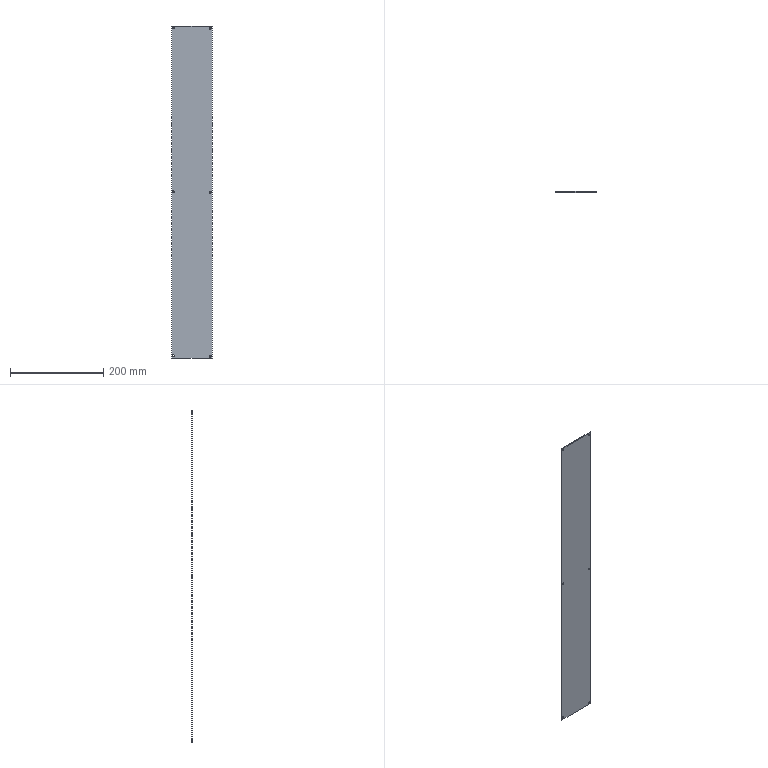Component | SolidWorks | ElectricalBoxCoverPlate2-1 | 1 solid | 18 faces | box 88 x 2 x 713 mm | volume 125337 mm3 | cylinder 12 | plane 6 | commonest cylinder face diameters 4 x12
build123d program:
from build123d import *

# Parameters (mm, degrees)
SKETCH1_W           = 713
SKETCH1_H           = 88
BOSS_EXTRUDE1_DEPTH = 2
SKETCH2_R           = 2
CUT_EXTRUDE1_DEPTH  = 2
LPATTERN1_COUNT     = 3
LPATTERN1_PITCH     = 352


with BuildPart() as part:
    # Sketch1 → Boss-Extrude1 (new body)
    with BuildSketch(Plane.XY):
        with Locations((280.981, -8.624)):
            Rectangle(SKETCH1_W, SKETCH1_H)
    extrude(amount=BOSS_EXTRUDE1_DEPTH)

    # Sketch2 → Cut-Extrude1 (cut)
    with BuildSketch(Plane.XY.offset(2)):
        with Locations((-71.519, 31.376)):
            Circle(SKETCH2_R)
        with Locations((-70.519, -47.624)):
            Circle(SKETCH2_R)
    cut_extrude1 = extrude(amount=-CUT_EXTRUDE1_DEPTH, mode=Mode.SUBTRACT)

    # LPattern1: Cut-Extrude1 ×3
    with Locations(*[(i * LPATTERN1_PITCH, 0, 0) for i in range(1, LPATTERN1_COUNT)]):
        add(cut_extrude1, mode=Mode.SUBTRACT)


solid = part.part

# Placed as in the assembly
solid = solid.moved(Location((311.826, 539.566, 414.962), (-90, 0, 90)))
STEP:
#1=COLOUR_RGB('',0.7922,0.8196,0.9333);
#2=FILL_AREA_STYLE_COLOUR('',#1);
#3=FILL_AREA_STYLE('',(#2));
#4=SURFACE_STYLE_FILL_AREA(#3);
#5=SURFACE_SIDE_STYLE('',(#4));
#6=SURFACE_STYLE_USAGE(.BOTH.,#5);
#7=PRESENTATION_STYLE_ASSIGNMENT((#6));
#8=CARTESIAN_POINT('',(14.152,21.243,-8.524));
#9=VERTEX_POINT('',#8);
#10=CARTESIAN_POINT('',(14.152,21.243,-8.682));
#11=VERTEX_POINT('',#10);
#12=CARTESIAN_POINT('',(14.152,21.243,-8.603));
#13=DIRECTION('',(0.,1.,0.));
#14=DIRECTION('',(0.,0.,-1.));
#15=AXIS2_PLACEMENT_3D('',#12,#13,#14);
#16=CIRCLE('',#15,0.07874);
#17=EDGE_CURVE('',#9,#11,#16,.T.);
#18=ORIENTED_EDGE('',*,*,#17,.F.);
#19=CARTESIAN_POINT('',(14.152,21.322,-8.524));
#20=VERTEX_POINT('',#19);
#21=CARTESIAN_POINT('',(14.152,21.243,-8.524));
#22=DIRECTION('',(0.,1.,0.));
#23=VECTOR('',#22,39.37);
#24=LINE('',#21,#23);
#25=EDGE_CURVE('',#9,#20,#24,.T.);
#26=ORIENTED_EDGE('',*,*,#25,.T.);
#27=CARTESIAN_POINT('',(14.152,21.322,-8.682));
#28=VERTEX_POINT('',#27);
#29=CARTESIAN_POINT('',(14.152,21.322,-8.603));
#30=DIRECTION('',(0.,1.,0.));
#31=DIRECTION('',(0.,0.,-1.));
#32=AXIS2_PLACEMENT_3D('',#29,#30,#31);
#33=CIRCLE('',#32,0.07874);
#34=EDGE_CURVE('',#20,#28,#33,.T.);
#35=ORIENTED_EDGE('',*,*,#34,.T.);
#36=CARTESIAN_POINT('',(14.152,21.243,-8.682));
#37=DIRECTION('',(0.,1.,0.));
#38=VECTOR('',#37,39.37);
#39=LINE('',#36,#38);
#40=EDGE_CURVE('',#11,#28,#39,.T.);
#41=ORIENTED_EDGE('',*,*,#40,.F.);
#42=EDGE_LOOP('',(#18,#26,#35,#41));
#43=FACE_OUTER_BOUND('',#42,.T.);
#44=CARTESIAN_POINT('',(14.152,21.243,-8.603));
#45=DIRECTION('',(0.,1.,0.));
#46=DIRECTION('',(0.,0.,-1.));
#47=AXIS2_PLACEMENT_3D('',#44,#45,#46);
#48=CYLINDRICAL_SURFACE('',#47,0.07874);
#49=ADVANCED_FACE('',(#43),#48,.F.);
#50=CARTESIAN_POINT('',(11.041,21.243,-8.485));
#51=VERTEX_POINT('',#50);
#52=CARTESIAN_POINT('',(11.041,21.243,-8.642));
#53=VERTEX_POINT('',#52);
#54=CARTESIAN_POINT('',(11.041,21.243,-8.564));
#55=DIRECTION('',(0.,1.,0.));
#56=DIRECTION('',(0.,0.,-1.));
#57=AXIS2_PLACEMENT_3D('',#54,#55,#56);
#58=CIRCLE('',#57,0.07874);
#59=EDGE_CURVE('',#51,#53,#58,.T.);
#60=ORIENTED_EDGE('',*,*,#59,.F.);
#61=CARTESIAN_POINT('',(11.041,21.322,-8.485));
#62=VERTEX_POINT('',#61);
#63=CARTESIAN_POINT('',(11.041,21.243,-8.485));
#64=DIRECTION('',(0.,1.,0.));
#65=VECTOR('',#64,39.37);
#66=LINE('',#63,#65);
#67=EDGE_CURVE('',#51,#62,#66,.T.);
#68=ORIENTED_EDGE('',*,*,#67,.T.);
#69=CARTESIAN_POINT('',(11.041,21.322,-8.642));
#70=VERTEX_POINT('',#69);
#71=CARTESIAN_POINT('',(11.041,21.322,-8.564));
#72=DIRECTION('',(0.,1.,0.));
#73=DIRECTION('',(0.,0.,-1.));
#74=AXIS2_PLACEMENT_3D('',#71,#72,#73);
#75=CIRCLE('',#74,0.07874);
#76=EDGE_CURVE('',#62,#70,#75,.T.);
#77=ORIENTED_EDGE('',*,*,#76,.T.);
#78=CARTESIAN_POINT('',(11.041,21.243,-8.642));
#79=DIRECTION('',(0.,1.,0.));
#80=VECTOR('',#79,39.37);
#81=LINE('',#78,#80);
#82=EDGE_CURVE('',#53,#70,#81,.T.);
#83=ORIENTED_EDGE('',*,*,#82,.F.);
#84=EDGE_LOOP('',(#60,#68,#77,#83));
#85=FACE_OUTER_BOUND('',#84,.T.);
#86=CARTESIAN_POINT('',(11.041,21.243,-8.564));
#87=DIRECTION('',(0.,1.,0.));
#88=DIRECTION('',(0.,0.,-1.));
#89=AXIS2_PLACEMENT_3D('',#86,#87,#88);
#90=CYLINDRICAL_SURFACE('',#89,0.07874);
#91=ADVANCED_FACE('',(#85),#90,.F.);
#92=CARTESIAN_POINT('',(14.152,21.243,5.334));
#93=VERTEX_POINT('',#92);
#94=CARTESIAN_POINT('',(14.152,21.243,5.176));
#95=VERTEX_POINT('',#94);
#96=CARTESIAN_POINT('',(14.152,21.243,5.255));
#97=DIRECTION('',(0.,1.,0.));
#98=DIRECTION('',(0.,0.,-1.));
#99=AXIS2_PLACEMENT_3D('',#96,#97,#98);
#100=CIRCLE('',#99,0.07874);
#101=EDGE_CURVE('',#93,#95,#100,.T.);
#102=ORIENTED_EDGE('',*,*,#101,.F.);
#103=CARTESIAN_POINT('',(14.152,21.322,5.334));
#104=VERTEX_POINT('',#103);
#105=CARTESIAN_POINT('',(14.152,21.243,5.334));
#106=DIRECTION('',(0.,1.,0.));
#107=VECTOR('',#106,39.37);
#108=LINE('',#105,#107);
#109=EDGE_CURVE('',#93,#104,#108,.T.);
#110=ORIENTED_EDGE('',*,*,#109,.T.);
#111=CARTESIAN_POINT('',(14.152,21.322,5.176));
#112=VERTEX_POINT('',#111);
#113=CARTESIAN_POINT('',(14.152,21.322,5.255));
#114=DIRECTION('',(0.,1.,0.));
#115=DIRECTION('',(0.,0.,-1.));
#116=AXIS2_PLACEMENT_3D('',#113,#114,#115);
#117=CIRCLE('',#116,0.07874);
#118=EDGE_CURVE('',#104,#112,#117,.T.);
#119=ORIENTED_EDGE('',*,*,#118,.T.);
#120=CARTESIAN_POINT('',(14.152,21.243,5.176));
#121=DIRECTION('',(0.,1.,0.));
#122=VECTOR('',#121,39.37);
#123=LINE('',#120,#122);
#124=EDGE_CURVE('',#95,#112,#123,.T.);
#125=ORIENTED_EDGE('',*,*,#124,.F.);
#126=EDGE_LOOP('',(#102,#110,#119,#125));
#127=FACE_OUTER_BOUND('',#126,.T.);
#128=CARTESIAN_POINT('',(14.152,21.243,5.255));
#129=DIRECTION('',(0.,1.,0.));
#130=DIRECTION('',(0.,0.,-1.));
#131=AXIS2_PLACEMENT_3D('',#128,#129,#130);
#132=CYLINDRICAL_SURFACE('',#131,0.07874);
#133=ADVANCED_FACE('',(#127),#132,.F.);
#134=CARTESIAN_POINT('',(11.041,21.243,5.373));
#135=VERTEX_POINT('',#134);
#136=CARTESIAN_POINT('',(11.041,21.243,5.216));
#137=VERTEX_POINT('',#136);
#138=CARTESIAN_POINT('',(11.041,21.243,5.295));
#139=DIRECTION('',(0.,1.,0.));
#140=DIRECTION('',(0.,0.,-1.));
#141=AXIS2_PLACEMENT_3D('',#138,#139,#140);
#142=CIRCLE('',#141,0.07874);
#143=EDGE_CURVE('',#135,#137,#142,.T.);
#144=ORIENTED_EDGE('',*,*,#143,.F.);
#145=CARTESIAN_POINT('',(11.041,21.322,5.373));
#146=VERTEX_POINT('',#145);
#147=CARTESIAN_POINT('',(11.041,21.243,5.373));
#148=DIRECTION('',(0.,1.,0.));
#149=VECTOR('',#148,39.37);
#150=LINE('',#147,#149);
#151=EDGE_CURVE('',#135,#146,#150,.T.);
#152=ORIENTED_EDGE('',*,*,#151,.T.);
#153=CARTESIAN_POINT('',(11.041,21.322,5.216));
#154=VERTEX_POINT('',#153);
#155=CARTESIAN_POINT('',(11.041,21.322,5.295));
#156=DIRECTION('',(0.,1.,0.));
#157=DIRECTION('',(0.,0.,-1.));
#158=AXIS2_PLACEMENT_3D('',#155,#156,#157);
#159=CIRCLE('',#158,0.07874);
#160=EDGE_CURVE('',#146,#154,#159,.T.);
#161=ORIENTED_EDGE('',*,*,#160,.T.);
#162=CARTESIAN_POINT('',(11.041,21.243,5.216));
#163=DIRECTION('',(0.,1.,0.));
#164=VECTOR('',#163,39.37);
#165=LINE('',#162,#164);
#166=EDGE_CURVE('',#137,#154,#165,.T.);
#167=ORIENTED_EDGE('',*,*,#166,.F.);
#168=EDGE_LOOP('',(#144,#152,#161,#167));
#169=FACE_OUTER_BOUND('',#168,.T.);
#170=CARTESIAN_POINT('',(11.041,21.243,5.295));
#171=DIRECTION('',(0.,1.,0.));
#172=DIRECTION('',(0.,0.,-1.));
#173=AXIS2_PLACEMENT_3D('',#170,#171,#172);
#174=CYLINDRICAL_SURFACE('',#173,0.07874);
#175=ADVANCED_FACE('',(#169),#174,.F.);
#176=CARTESIAN_POINT('',(14.152,21.243,19.192));
#177=VERTEX_POINT('',#176);
#178=CARTESIAN_POINT('',(14.152,21.243,19.035));
#179=VERTEX_POINT('',#178);
#180=CARTESIAN_POINT('',(14.152,21.243,19.113));
#181=DIRECTION('',(0.,1.,0.));
#182=DIRECTION('',(0.,0.,-1.));
#183=AXIS2_PLACEMENT_3D('',#180,#181,#182);
#184=CIRCLE('',#183,0.07874);
#185=EDGE_CURVE('',#177,#179,#184,.T.);
#186=ORIENTED_EDGE('',*,*,#185,.F.);
#187=CARTESIAN_POINT('',(14.152,21.322,19.192));
#188=VERTEX_POINT('',#187);
#189=CARTESIAN_POINT('',(14.152,21.243,19.192));
#190=DIRECTION('',(0.,1.,0.));
#191=VECTOR('',#190,39.37);
#192=LINE('',#189,#191);
#193=EDGE_CURVE('',#177,#188,#192,.T.);
#194=ORIENTED_EDGE('',*,*,#193,.T.);
#195=CARTESIAN_POINT('',(14.152,21.322,19.035));
#196=VERTEX_POINT('',#195);
#197=CARTESIAN_POINT('',(14.152,21.322,19.113));
#198=DIRECTION('',(0.,1.,0.));
#199=DIRECTION('',(0.,0.,-1.));
#200=AXIS2_PLACEMENT_3D('',#197,#198,#199);
#201=CIRCLE('',#200,0.07874);
#202=EDGE_CURVE('',#188,#196,#201,.T.);
#203=ORIENTED_EDGE('',*,*,#202,.T.);
#204=CARTESIAN_POINT('',(14.152,21.243,19.035));
#205=DIRECTION('',(0.,1.,0.));
#206=VECTOR('',#205,39.37);
#207=LINE('',#204,#206);
#208=EDGE_CURVE('',#179,#196,#207,.T.);
#209=ORIENTED_EDGE('',*,*,#208,.F.);
#210=EDGE_LOOP('',(#186,#194,#203,#209));
#211=FACE_OUTER_BOUND('',#210,.T.);
#212=CARTESIAN_POINT('',(14.152,21.243,19.113));
#213=DIRECTION('',(0.,1.,0.));
#214=DIRECTION('',(0.,0.,-1.));
#215=AXIS2_PLACEMENT_3D('',#212,#213,#214);
#216=CYLINDRICAL_SURFACE('',#215,0.07874);
#217=ADVANCED_FACE('',(#211),#216,.F.);
#218=CARTESIAN_POINT('',(11.041,21.243,19.232));
#219=VERTEX_POINT('',#218);
#220=CARTESIAN_POINT('',(11.041,21.243,19.074));
#221=VERTEX_POINT('',#220);
#222=CARTESIAN_POINT('',(11.041,21.243,19.153));
#223=DIRECTION('',(0.,1.,0.));
#224=DIRECTION('',(0.,0.,-1.));
#225=AXIS2_PLACEMENT_3D('',#222,#223,#224);
#226=CIRCLE('',#225,0.07874);
#227=EDGE_CURVE('',#219,#221,#226,.T.);
#228=ORIENTED_EDGE('',*,*,#227,.F.);
#229=CARTESIAN_POINT('',(11.041,21.322,19.232));
#230=VERTEX_POINT('',#229);
#231=CARTESIAN_POINT('',(11.041,21.243,19.232));
#232=DIRECTION('',(0.,1.,0.));
#233=VECTOR('',#232,39.37);
#234=LINE('',#231,#233);
#235=EDGE_CURVE('',#219,#230,#234,.T.);
#236=ORIENTED_EDGE('',*,*,#235,.T.);
#237=CARTESIAN_POINT('',(11.041,21.322,19.074));
#238=VERTEX_POINT('',#237);
#239=CARTESIAN_POINT('',(11.041,21.322,19.153));
#240=DIRECTION('',(0.,1.,0.));
#241=DIRECTION('',(0.,0.,-1.));
#242=AXIS2_PLACEMENT_3D('',#239,#240,#241);
#243=CIRCLE('',#242,0.07874);
#244=EDGE_CURVE('',#230,#238,#243,.T.);
#245=ORIENTED_EDGE('',*,*,#244,.T.);
#246=CARTESIAN_POINT('',(11.041,21.243,19.074));
#247=DIRECTION('',(0.,1.,0.));
#248=VECTOR('',#247,39.37);
#249=LINE('',#246,#248);
#250=EDGE_CURVE('',#221,#238,#249,.T.);
#251=ORIENTED_EDGE('',*,*,#250,.F.);
#252=EDGE_LOOP('',(#228,#236,#245,#251));
#253=FACE_OUTER_BOUND('',#252,.T.);
#254=CARTESIAN_POINT('',(11.041,21.243,19.153));
#255=DIRECTION('',(0.,1.,0.));
#256=DIRECTION('',(0.,0.,-1.));
#257=AXIS2_PLACEMENT_3D('',#254,#255,#256);
#258=CYLINDRICAL_SURFACE('',#257,0.07874);
#259=ADVANCED_FACE('',(#253),#258,.F.);
#260=CARTESIAN_POINT('',(10.884,21.243,19.31));
#261=VERTEX_POINT('',#260);
#262=CARTESIAN_POINT('',(14.348,21.243,19.31));
#263=VERTEX_POINT('',#262);
#264=CARTESIAN_POINT('',(10.884,21.243,19.31));
#265=DIRECTION('',(1.,0.,-0.));
#266=VECTOR('',#265,39.37);
#267=LINE('',#264,#266);
#268=EDGE_CURVE('',#261,#263,#267,.T.);
#269=ORIENTED_EDGE('',*,*,#268,.T.);
#270=CARTESIAN_POINT('',(14.348,21.322,19.31));
#271=VERTEX_POINT('',#270);
#272=CARTESIAN_POINT('',(14.348,21.322,19.31));
#273=DIRECTION('',(0.,-1.,-0.));
#274=VECTOR('',#273,39.37);
#275=LINE('',#272,#274);
#276=EDGE_CURVE('',#271,#263,#275,.T.);
#277=ORIENTED_EDGE('',*,*,#276,.F.);
#278=CARTESIAN_POINT('',(10.884,21.322,19.31));
#279=VERTEX_POINT('',#278);
#280=CARTESIAN_POINT('',(10.884,21.322,19.31));
#281=DIRECTION('',(1.,0.,-0.));
#282=VECTOR('',#281,39.37);
#283=LINE('',#280,#282);
#284=EDGE_CURVE('',#279,#271,#283,.T.);
#285=ORIENTED_EDGE('',*,*,#284,.F.);
#286=CARTESIAN_POINT('',(10.884,21.322,19.31));
#287=DIRECTION('',(0.,-1.,-0.));
#288=VECTOR('',#287,39.37);
#289=LINE('',#286,#288);
#290=EDGE_CURVE('',#279,#261,#289,.T.);
#291=ORIENTED_EDGE('',*,*,#290,.T.);
#292=EDGE_LOOP('',(#269,#277,#285,#291));
#293=FACE_OUTER_BOUND('',#292,.T.);
#294=CARTESIAN_POINT('',(10.884,21.322,19.31));
#295=DIRECTION('',(-0.,0.,-1.));
#296=DIRECTION('',(-1.,-0.,0.));
#297=AXIS2_PLACEMENT_3D('',#294,#295,#296);
#298=PLANE('',#297);
#299=ADVANCED_FACE('',(#293),#298,.F.);
#300=CARTESIAN_POINT('',(14.348,21.243,-8.761));
#301=VERTEX_POINT('',#300);
#302=CARTESIAN_POINT('',(14.348,21.243,19.31));
#303=DIRECTION('',(-0.,0.,-1.));
#304=VECTOR('',#303,39.37);
#305=LINE('',#302,#304);
#306=EDGE_CURVE('',#263,#301,#305,.T.);
#307=ORIENTED_EDGE('',*,*,#306,.T.);
#308=CARTESIAN_POINT('',(14.348,21.322,-8.761));
#309=VERTEX_POINT('',#308);
#310=CARTESIAN_POINT('',(14.348,21.322,-8.761));
#311=DIRECTION('',(0.,-1.,-0.));
#312=VECTOR('',#311,39.37);
#313=LINE('',#310,#312);
#314=EDGE_CURVE('',#309,#301,#313,.T.);
#315=ORIENTED_EDGE('',*,*,#314,.F.);
#316=CARTESIAN_POINT('',(14.348,21.322,19.31));
#317=DIRECTION('',(-0.,0.,-1.));
#318=VECTOR('',#317,39.37);
#319=LINE('',#316,#318);
#320=EDGE_CURVE('',#271,#309,#319,.T.);
#321=ORIENTED_EDGE('',*,*,#320,.F.);
#322=ORIENTED_EDGE('',*,*,#276,.T.);
#323=EDGE_LOOP('',(#307,#315,#321,#322));
#324=FACE_OUTER_BOUND('',#323,.T.);
#325=CARTESIAN_POINT('',(14.348,21.322,19.31));
#326=DIRECTION('',(-1.,-0.,0.));
#327=DIRECTION('',(0.,1.,0.));
#328=AXIS2_PLACEMENT_3D('',#325,#326,#327);
#329=PLANE('',#328);
#330=ADVANCED_FACE('',(#324),#329,.F.);
#331=CARTESIAN_POINT('',(10.884,21.243,-8.761));
#332=VERTEX_POINT('',#331);
#333=CARTESIAN_POINT('',(10.884,21.243,-8.761));
#334=DIRECTION('',(-1.,-0.,0.));
#335=VECTOR('',#334,39.37);
#336=LINE('',#333,#335);
#337=EDGE_CURVE('',#301,#332,#336,.T.);
#338=ORIENTED_EDGE('',*,*,#337,.T.);
#339=CARTESIAN_POINT('',(10.884,21.322,-8.761));
#340=VERTEX_POINT('',#339);
#341=CARTESIAN_POINT('',(10.884,21.322,-8.761));
#342=DIRECTION('',(0.,-1.,-0.));
#343=VECTOR('',#342,39.37);
#344=LINE('',#341,#343);
#345=EDGE_CURVE('',#340,#332,#344,.T.);
#346=ORIENTED_EDGE('',*,*,#345,.F.);
#347=CARTESIAN_POINT('',(10.884,21.322,-8.761));
#348=DIRECTION('',(-1.,-0.,0.));
#349=VECTOR('',#348,39.37);
#350=LINE('',#347,#349);
#351=EDGE_CURVE('',#309,#340,#350,.T.);
#352=ORIENTED_EDGE('',*,*,#351,.F.);
#353=ORIENTED_EDGE('',*,*,#314,.T.);
#354=EDGE_LOOP('',(#338,#346,#352,#353));
#355=FACE_OUTER_BOUND('',#354,.T.);
#356=CARTESIAN_POINT('',(10.884,21.322,-8.761));
#357=DIRECTION('',(0.,-0.,1.));
#358=DIRECTION('',(0.,1.,0.));
#359=AXIS2_PLACEMENT_3D('',#356,#357,#358);
#360=PLANE('',#359);
#361=ADVANCED_FACE('',(#355),#360,.F.);
#362=CARTESIAN_POINT('',(10.884,21.243,19.31));
#363=DIRECTION('',(0.,-0.,1.));
#364=VECTOR('',#363,39.37);
#365=LINE('',#362,#364);
#366=EDGE_CURVE('',#332,#261,#365,.T.);
#367=ORIENTED_EDGE('',*,*,#366,.T.);
#368=ORIENTED_EDGE('',*,*,#290,.F.);
#369=CARTESIAN_POINT('',(10.884,21.322,19.31));
#370=DIRECTION('',(0.,-0.,1.));
#371=VECTOR('',#370,39.37);
#372=LINE('',#369,#371);
#373=EDGE_CURVE('',#340,#279,#372,.T.);
#374=ORIENTED_EDGE('',*,*,#373,.F.);
#375=ORIENTED_EDGE('',*,*,#345,.T.);
#376=EDGE_LOOP('',(#367,#368,#374,#375));
#377=FACE_OUTER_BOUND('',#376,.T.);
#378=CARTESIAN_POINT('',(10.884,21.322,19.31));
#379=DIRECTION('',(1.,0.,-0.));
#380=DIRECTION('',(0.,-1.,-0.));
#381=AXIS2_PLACEMENT_3D('',#378,#379,#380);
#382=PLANE('',#381);
#383=ADVANCED_FACE('',(#377),#382,.F.);
#384=CARTESIAN_POINT('',(14.152,21.322,5.255));
#385=DIRECTION('',(0.,1.,0.));
#386=DIRECTION('',(0.,0.,-1.));
#387=AXIS2_PLACEMENT_3D('',#384,#385,#386);
#388=CIRCLE('',#387,0.07874);
#389=EDGE_CURVE('',#112,#104,#388,.T.);
#390=ORIENTED_EDGE('',*,*,#389,.F.);
#391=ORIENTED_EDGE('',*,*,#118,.F.);
#392=EDGE_LOOP('',(#390,#391));
#393=FACE_BOUND('',#392,.T.);
#394=CARTESIAN_POINT('',(11.041,21.322,5.295));
#395=DIRECTION('',(0.,1.,0.));
#396=DIRECTION('',(0.,0.,-1.));
#397=AXIS2_PLACEMENT_3D('',#394,#395,#396);
#398=CIRCLE('',#397,0.07874);
#399=EDGE_CURVE('',#154,#146,#398,.T.);
#400=ORIENTED_EDGE('',*,*,#399,.F.);
#401=ORIENTED_EDGE('',*,*,#160,.F.);
#402=EDGE_LOOP('',(#400,#401));
#403=FACE_BOUND('',#402,.T.);
#404=CARTESIAN_POINT('',(14.152,21.322,19.113));
#405=DIRECTION('',(0.,1.,0.));
#406=DIRECTION('',(0.,0.,-1.));
#407=AXIS2_PLACEMENT_3D('',#404,#405,#406);
#408=CIRCLE('',#407,0.07874);
#409=EDGE_CURVE('',#196,#188,#408,.T.);
#410=ORIENTED_EDGE('',*,*,#409,.F.);
#411=ORIENTED_EDGE('',*,*,#202,.F.);
#412=EDGE_LOOP('',(#410,#411));
#413=FACE_BOUND('',#412,.T.);
#414=CARTESIAN_POINT('',(11.041,21.322,19.153));
#415=DIRECTION('',(0.,1.,0.));
#416=DIRECTION('',(0.,0.,-1.));
#417=AXIS2_PLACEMENT_3D('',#414,#415,#416);
#418=CIRCLE('',#417,0.07874);
#419=EDGE_CURVE('',#238,#230,#418,.T.);
#420=ORIENTED_EDGE('',*,*,#419,.F.);
#421=ORIENTED_EDGE('',*,*,#244,.F.);
#422=EDGE_LOOP('',(#420,#421));
#423=FACE_BOUND('',#422,.T.);
#424=ORIENTED_EDGE('',*,*,#284,.T.);
#425=ORIENTED_EDGE('',*,*,#320,.T.);
#426=ORIENTED_EDGE('',*,*,#351,.T.);
#427=ORIENTED_EDGE('',*,*,#373,.T.);
#428=EDGE_LOOP('',(#424,#425,#426,#427));
#429=FACE_OUTER_BOUND('',#428,.T.);
#430=CARTESIAN_POINT('',(11.041,21.322,-8.564));
#431=DIRECTION('',(0.,1.,0.));
#432=DIRECTION('',(0.,0.,-1.));
#433=AXIS2_PLACEMENT_3D('',#430,#431,#432);
#434=CIRCLE('',#433,0.07874);
#435=EDGE_CURVE('',#70,#62,#434,.T.);
#436=ORIENTED_EDGE('',*,*,#435,.F.);
#437=ORIENTED_EDGE('',*,*,#76,.F.);
#438=EDGE_LOOP('',(#436,#437));
#439=FACE_BOUND('',#438,.T.);
#440=CARTESIAN_POINT('',(14.152,21.322,-8.603));
#441=DIRECTION('',(0.,1.,0.));
#442=DIRECTION('',(0.,0.,-1.));
#443=AXIS2_PLACEMENT_3D('',#440,#441,#442);
#444=CIRCLE('',#443,0.07874);
#445=EDGE_CURVE('',#28,#20,#444,.T.);
#446=ORIENTED_EDGE('',*,*,#445,.F.);
#447=ORIENTED_EDGE('',*,*,#34,.F.);
#448=EDGE_LOOP('',(#446,#447));
#449=FACE_BOUND('',#448,.T.);
#450=CARTESIAN_POINT('',(12.277,21.322,16.337));
#451=DIRECTION('',(0.,1.,0.));
#452=DIRECTION('',(-0.,0.,-1.));
#453=AXIS2_PLACEMENT_3D('',#450,#451,#452);
#454=PLANE('',#453);
#455=ADVANCED_FACE('',(#393,#403,#413,#423,#429,#439,#449),#454,.T.);
#456=CARTESIAN_POINT('',(14.152,21.243,5.255));
#457=DIRECTION('',(0.,1.,0.));
#458=DIRECTION('',(0.,0.,-1.));
#459=AXIS2_PLACEMENT_3D('',#456,#457,#458);
#460=CIRCLE('',#459,0.07874);
#461=EDGE_CURVE('',#95,#93,#460,.T.);
#462=ORIENTED_EDGE('',*,*,#461,.T.);
#463=ORIENTED_EDGE('',*,*,#101,.T.);
#464=EDGE_LOOP('',(#462,#463));
#465=FACE_BOUND('',#464,.T.);
#466=CARTESIAN_POINT('',(11.041,21.243,5.295));
#467=DIRECTION('',(0.,1.,0.));
#468=DIRECTION('',(0.,0.,-1.));
#469=AXIS2_PLACEMENT_3D('',#466,#467,#468);
#470=CIRCLE('',#469,0.07874);
#471=EDGE_CURVE('',#137,#135,#470,.T.);
#472=ORIENTED_EDGE('',*,*,#471,.T.);
#473=ORIENTED_EDGE('',*,*,#143,.T.);
#474=EDGE_LOOP('',(#472,#473));
#475=FACE_BOUND('',#474,.T.);
#476=CARTESIAN_POINT('',(14.152,21.243,19.113));
#477=DIRECTION('',(0.,1.,0.));
#478=DIRECTION('',(0.,0.,-1.));
#479=AXIS2_PLACEMENT_3D('',#476,#477,#478);
#480=CIRCLE('',#479,0.07874);
#481=EDGE_CURVE('',#179,#177,#480,.T.);
#482=ORIENTED_EDGE('',*,*,#481,.T.);
#483=ORIENTED_EDGE('',*,*,#185,.T.);
#484=EDGE_LOOP('',(#482,#483));
#485=FACE_BOUND('',#484,.T.);
#486=CARTESIAN_POINT('',(11.041,21.243,19.153));
#487=DIRECTION('',(0.,1.,0.));
#488=DIRECTION('',(0.,0.,-1.));
#489=AXIS2_PLACEMENT_3D('',#486,#487,#488);
#490=CIRCLE('',#489,0.07874);
#491=EDGE_CURVE('',#221,#219,#490,.T.);
#492=ORIENTED_EDGE('',*,*,#491,.T.);
#493=ORIENTED_EDGE('',*,*,#227,.T.);
#494=EDGE_LOOP('',(#492,#493));
#495=FACE_BOUND('',#494,.T.);
#496=ORIENTED_EDGE('',*,*,#268,.F.);
#497=ORIENTED_EDGE('',*,*,#366,.F.);
#498=ORIENTED_EDGE('',*,*,#337,.F.);
#499=ORIENTED_EDGE('',*,*,#306,.F.);
#500=EDGE_LOOP('',(#496,#497,#498,#499));
#501=FACE_OUTER_BOUND('',#500,.T.);
#502=CARTESIAN_POINT('',(11.041,21.243,-8.564));
#503=DIRECTION('',(0.,1.,0.));
#504=DIRECTION('',(0.,0.,-1.));
#505=AXIS2_PLACEMENT_3D('',#502,#503,#504);
#506=CIRCLE('',#505,0.07874);
#507=EDGE_CURVE('',#53,#51,#506,.T.);
#508=ORIENTED_EDGE('',*,*,#507,.T.);
#509=ORIENTED_EDGE('',*,*,#59,.T.);
#510=EDGE_LOOP('',(#508,#509));
#511=FACE_BOUND('',#510,.T.);
#512=CARTESIAN_POINT('',(14.152,21.243,-8.603));
#513=DIRECTION('',(0.,1.,0.));
#514=DIRECTION('',(0.,0.,-1.));
#515=AXIS2_PLACEMENT_3D('',#512,#513,#514);
#516=CIRCLE('',#515,0.07874);
#517=EDGE_CURVE('',#11,#9,#516,.T.);
#518=ORIENTED_EDGE('',*,*,#517,.T.);
#519=ORIENTED_EDGE('',*,*,#17,.T.);
#520=EDGE_LOOP('',(#518,#519));
#521=FACE_BOUND('',#520,.T.);
#522=CARTESIAN_POINT('',(12.277,21.243,16.337));
#523=DIRECTION('',(0.,1.,0.));
#524=DIRECTION('',(-0.,0.,-1.));
#525=AXIS2_PLACEMENT_3D('',#522,#523,#524);
#526=PLANE('',#525);
#527=ADVANCED_FACE('',(#465,#475,#485,#495,#501,#511,#521),#526,.F.);
#528=ORIENTED_EDGE('',*,*,#235,.F.);
#529=ORIENTED_EDGE('',*,*,#491,.F.);
#530=ORIENTED_EDGE('',*,*,#250,.T.);
#531=ORIENTED_EDGE('',*,*,#419,.T.);
#532=EDGE_LOOP('',(#528,#529,#530,#531));
#533=FACE_OUTER_BOUND('',#532,.T.);
#534=CARTESIAN_POINT('',(11.041,21.243,19.153));
#535=DIRECTION('',(0.,1.,0.));
#536=DIRECTION('',(0.,0.,-1.));
#537=AXIS2_PLACEMENT_3D('',#534,#535,#536);
#538=CYLINDRICAL_SURFACE('',#537,0.07874);
#539=ADVANCED_FACE('',(#533),#538,.F.);
#540=ORIENTED_EDGE('',*,*,#193,.F.);
#541=ORIENTED_EDGE('',*,*,#481,.F.);
#542=ORIENTED_EDGE('',*,*,#208,.T.);
#543=ORIENTED_EDGE('',*,*,#409,.T.);
#544=EDGE_LOOP('',(#540,#541,#542,#543));
#545=FACE_OUTER_BOUND('',#544,.T.);
#546=CARTESIAN_POINT('',(14.152,21.243,19.113));
#547=DIRECTION('',(0.,1.,0.));
#548=DIRECTION('',(0.,0.,-1.));
#549=AXIS2_PLACEMENT_3D('',#546,#547,#548);
#550=CYLINDRICAL_SURFACE('',#549,0.07874);
#551=ADVANCED_FACE('',(#545),#550,.F.);
#552=ORIENTED_EDGE('',*,*,#151,.F.);
#553=ORIENTED_EDGE('',*,*,#471,.F.);
#554=ORIENTED_EDGE('',*,*,#166,.T.);
#555=ORIENTED_EDGE('',*,*,#399,.T.);
#556=EDGE_LOOP('',(#552,#553,#554,#555));
#557=FACE_OUTER_BOUND('',#556,.T.);
#558=CARTESIAN_POINT('',(11.041,21.243,5.295));
#559=DIRECTION('',(0.,1.,0.));
#560=DIRECTION('',(0.,0.,-1.));
#561=AXIS2_PLACEMENT_3D('',#558,#559,#560);
#562=CYLINDRICAL_SURFACE('',#561,0.07874);
#563=ADVANCED_FACE('',(#557),#562,.F.);
#564=ORIENTED_EDGE('',*,*,#109,.F.);
#565=ORIENTED_EDGE('',*,*,#461,.F.);
#566=ORIENTED_EDGE('',*,*,#124,.T.);
#567=ORIENTED_EDGE('',*,*,#389,.T.);
#568=EDGE_LOOP('',(#564,#565,#566,#567));
#569=FACE_OUTER_BOUND('',#568,.T.);
#570=CARTESIAN_POINT('',(14.152,21.243,5.255));
#571=DIRECTION('',(0.,1.,0.));
#572=DIRECTION('',(0.,0.,-1.));
#573=AXIS2_PLACEMENT_3D('',#570,#571,#572);
#574=CYLINDRICAL_SURFACE('',#573,0.07874);
#575=ADVANCED_FACE('',(#569),#574,.F.);
#576=ORIENTED_EDGE('',*,*,#67,.F.);
#577=ORIENTED_EDGE('',*,*,#507,.F.);
#578=ORIENTED_EDGE('',*,*,#82,.T.);
#579=ORIENTED_EDGE('',*,*,#435,.T.);
#580=EDGE_LOOP('',(#576,#577,#578,#579));
#581=FACE_OUTER_BOUND('',#580,.T.);
#582=CARTESIAN_POINT('',(11.041,21.243,-8.564));
#583=DIRECTION('',(0.,1.,0.));
#584=DIRECTION('',(0.,0.,-1.));
#585=AXIS2_PLACEMENT_3D('',#582,#583,#584);
#586=CYLINDRICAL_SURFACE('',#585,0.07874);
#587=ADVANCED_FACE('',(#581),#586,.F.);
#588=ORIENTED_EDGE('',*,*,#25,.F.);
#589=ORIENTED_EDGE('',*,*,#517,.F.);
#590=ORIENTED_EDGE('',*,*,#40,.T.);
#591=ORIENTED_EDGE('',*,*,#445,.T.);
#592=EDGE_LOOP('',(#588,#589,#590,#591));
#593=FACE_OUTER_BOUND('',#592,.T.);
#594=CARTESIAN_POINT('',(14.152,21.243,-8.603));
#595=DIRECTION('',(0.,1.,0.));
#596=DIRECTION('',(0.,0.,-1.));
#597=AXIS2_PLACEMENT_3D('',#594,#595,#596);
#598=CYLINDRICAL_SURFACE('',#597,0.07874);
#599=ADVANCED_FACE('',(#593),#598,.F.);
#600=CLOSED_SHELL('',(#49,#91,#133,#175,#217,#259,#299,#330,#361,#383,#455,#527,#539,#551,#563,#575,#587,#599));
#601=MANIFOLD_SOLID_BREP('',#600);
#602=STYLED_ITEM('',(#7),#601);
#603=PRESENTATION_LAYER_ASSIGNMENT('','',(#602));
#604=(LENGTH_UNIT()NAMED_UNIT(*)SI_UNIT($,.METRE.));
#605=LENGTH_MEASURE_WITH_UNIT(LENGTH_MEASURE(0.0254),#604);
#606=DIMENSIONAL_EXPONENTS(1.,0.,0.,0.,0.,0.,0.);
#607=(CONVERSION_BASED_UNIT('',#605)LENGTH_UNIT()NAMED_UNIT(#606));
#608=UNCERTAINTY_MEASURE_WITH_UNIT(LENGTH_MEASURE(0.00001),#607,'','');
#609=(NAMED_UNIT(*)PLANE_ANGLE_UNIT()SI_UNIT($,.RADIAN.));
#610=(NAMED_UNIT(*)SI_UNIT($,.STERADIAN.)SOLID_ANGLE_UNIT());
#611=(GEOMETRIC_REPRESENTATION_CONTEXT(3)GLOBAL_UNCERTAINTY_ASSIGNED_CONTEXT((#608))GLOBAL_UNIT_ASSIGNED_CONTEXT((#607,#609,#610))REPRESENTATION_CONTEXT('',''));
#612=MECHANICAL_DESIGN_GEOMETRIC_PRESENTATION_REPRESENTATION('',(#602),#611);
#613=CARTESIAN_POINT('',(0.,0.,0.));
#614=DIRECTION('',(0.,0.,1.));
#615=DIRECTION('',(1.,0.,0.));
#616=AXIS2_PLACEMENT_3D('',#613,#614,#615);
#617=(LENGTH_UNIT()NAMED_UNIT(*)SI_UNIT($,.METRE.));
#618=LENGTH_MEASURE_WITH_UNIT(LENGTH_MEASURE(0.0254),#617);
#619=DIMENSIONAL_EXPONENTS(1.,0.,0.,0.,0.,0.,0.);
#620=(CONVERSION_BASED_UNIT('',#618)LENGTH_UNIT()NAMED_UNIT(#619));
#621=UNCERTAINTY_MEASURE_WITH_UNIT(LENGTH_MEASURE(0.00001),#620,'','');
#622=(NAMED_UNIT(*)PLANE_ANGLE_UNIT()SI_UNIT($,.RADIAN.));
#623=(NAMED_UNIT(*)SI_UNIT($,.STERADIAN.)SOLID_ANGLE_UNIT());
#624=(GEOMETRIC_REPRESENTATION_CONTEXT(3)GLOBAL_UNCERTAINTY_ASSIGNED_CONTEXT((#621))GLOBAL_UNIT_ASSIGNED_CONTEXT((#620,#622,#623))REPRESENTATION_CONTEXT('',''));
#625=ADVANCED_BREP_SHAPE_REPRESENTATION('',(#601,#616),#624);